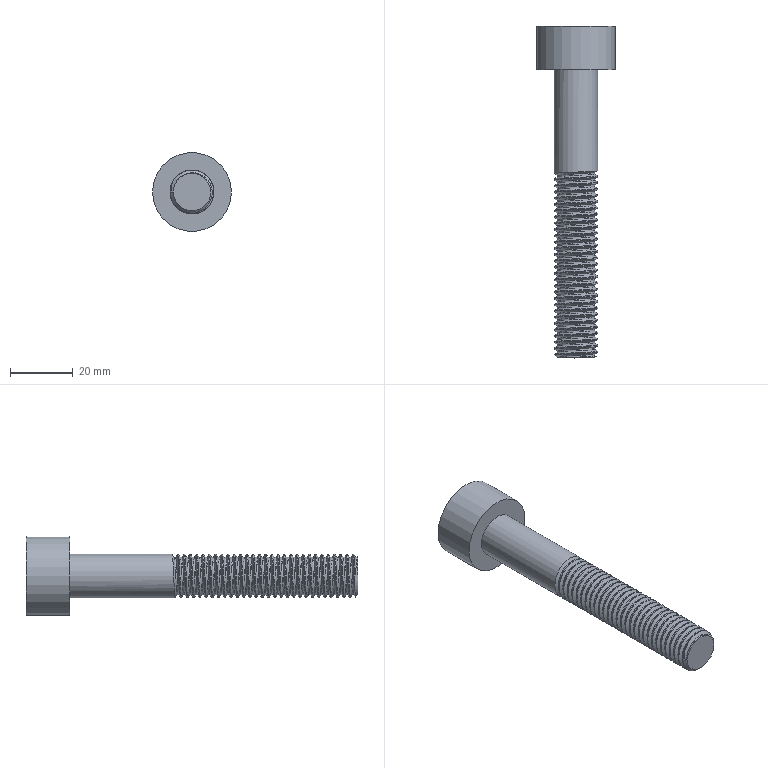Component | NX | ALLINE_SCREW_M14_SUP_2_SUP1_2 | 1 solid | 47 faces | volume 18629 mm3 | cylinder 32 | plane 12 | spline 2 | cone 1 | commonest cylinder face diameters 14 x30 25.2 x1 12 x1